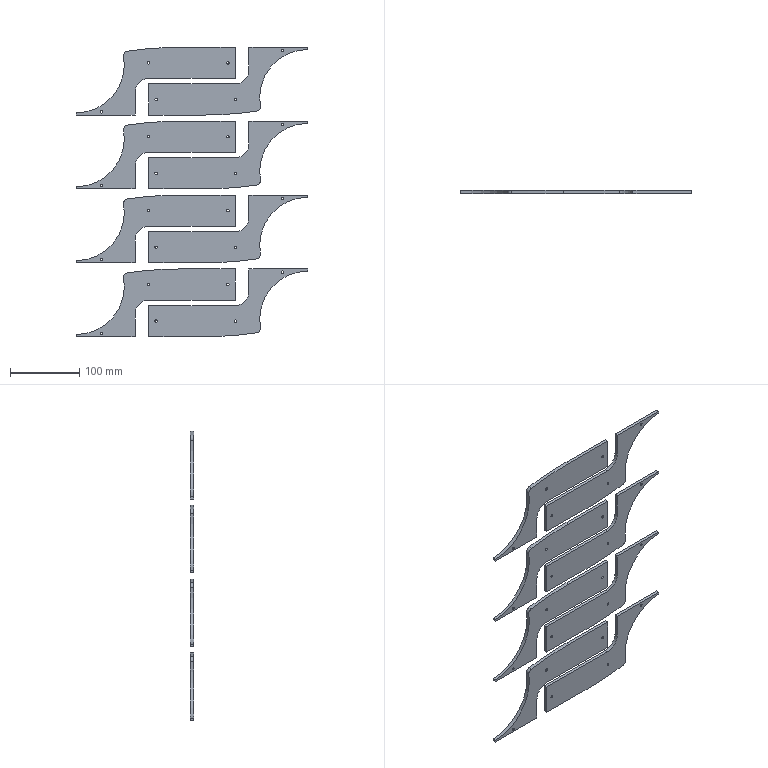CAM job | Mastercam | mm | 4 operations | part box 335 x 5 x 419
1. Contour (Ramp) | 3 - 3 平铣刀
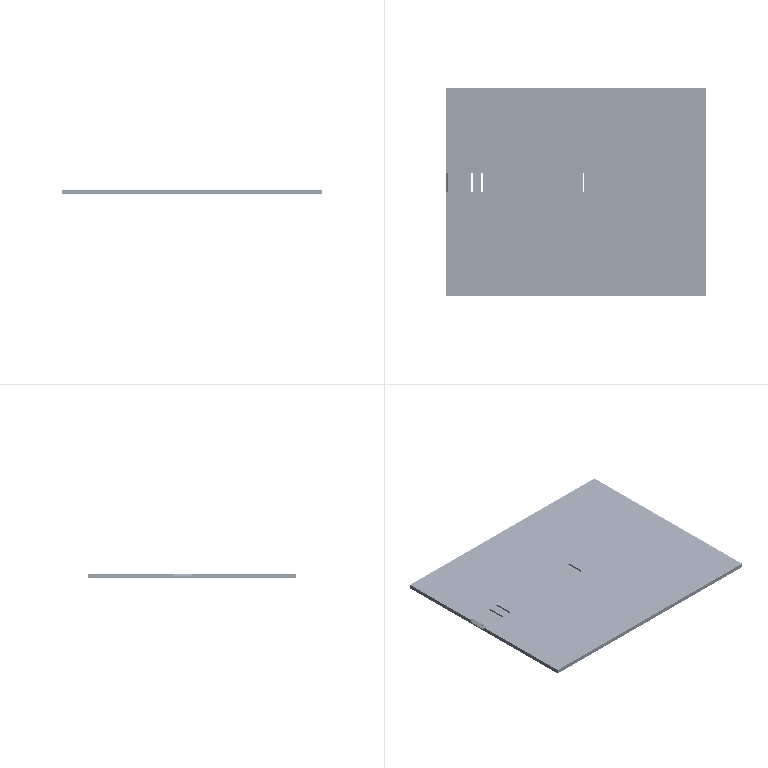2. Drill/Counterbore | 7 - 4 倒角刀
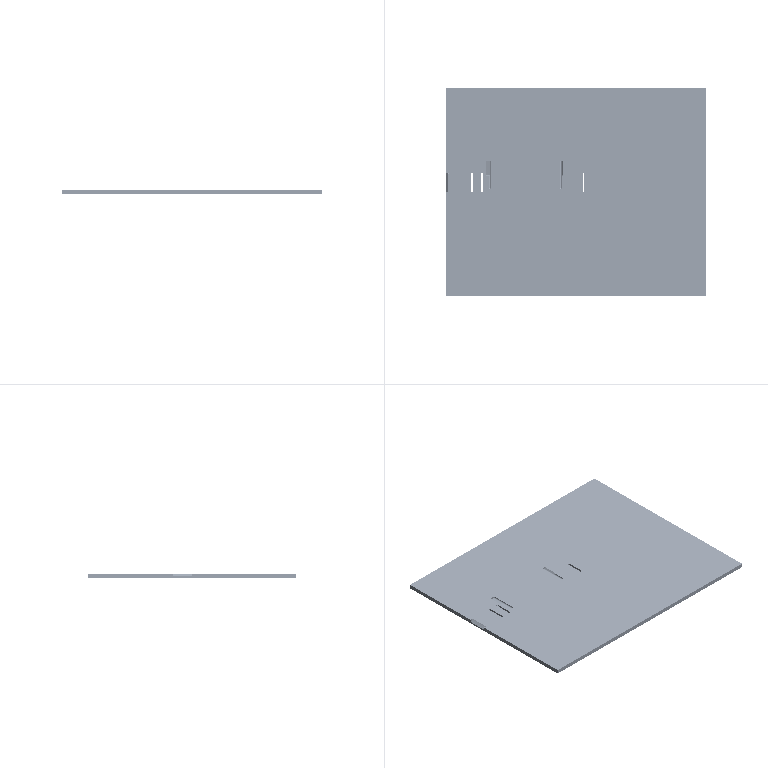3. Contour (2D chamfer) | 7 - 4 倒角刀
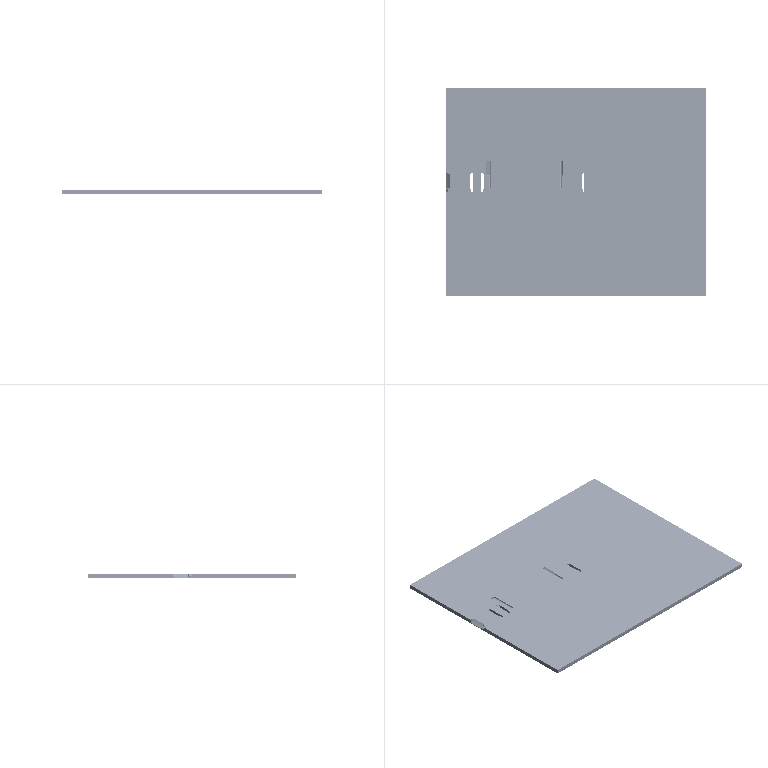4. Contour (Ramp) | 2 - 2 平铣刀